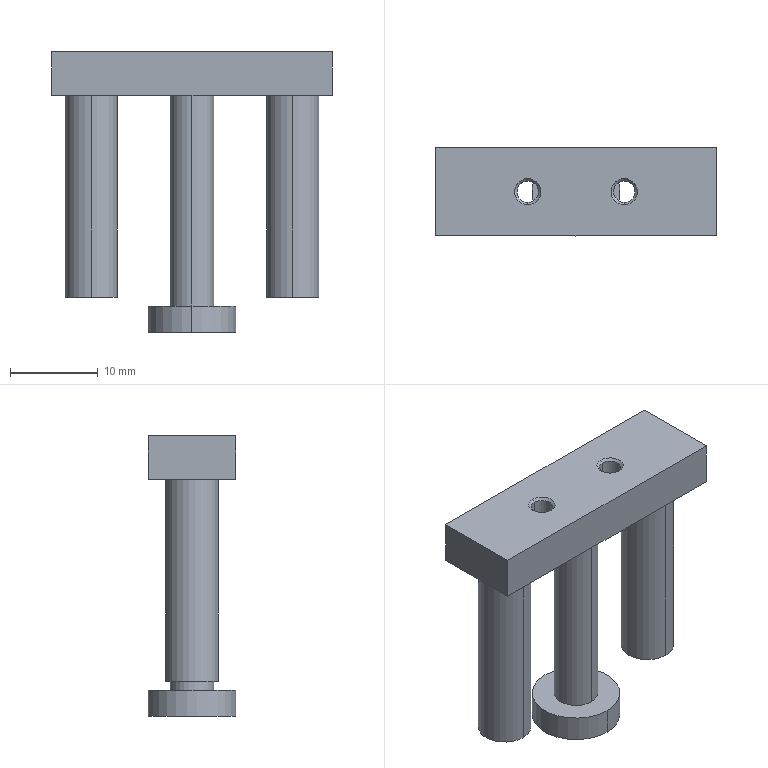Component | SolidWorks | MGJ10-15-1_2-11-1 | 1 solid | 30 faces | box 32 x 10 x 32 mm | volume 3559 mm3 | cylinder 12 | plane 10 | cone 8 | commonest cylinder face diameters 2.459 x4 6 x4 5 x2 10 x2
STEP:
#1=CARTESIAN_POINT('',(-0.4599,-4.569,-11.27));
#2=VERTEX_POINT('',#1);
#3=CARTESIAN_POINT('',(-0.4599,-4.665,-11.27));
#4=VERTEX_POINT('',#3);
#5=CARTESIAN_POINT('',(-0.4599,-4.617,-11.27));
#6=DIRECTION('',(0.,-0.,1.));
#7=DIRECTION('',(1.,0.,-0.));
#8=AXIS2_PLACEMENT_3D('',#5,#6,#7);
#9=CIRCLE('',#8,0.04841);
#10=EDGE_CURVE('',#2,#4,#9,.T.);
#11=ORIENTED_EDGE('',*,*,#10,.F.);
#12=CARTESIAN_POINT('',(-0.4599,-4.558,-11.259));
#13=VERTEX_POINT('',#12);
#14=CARTESIAN_POINT('',(-0.4599,-4.558,-11.259));
#15=DIRECTION('',(0.,0.7071,0.7071));
#16=VECTOR('',#15,39.37);
#17=LINE('',#14,#16);
#18=EDGE_CURVE('',#2,#13,#17,.T.);
#19=ORIENTED_EDGE('',*,*,#18,.T.);
#20=CARTESIAN_POINT('',(-0.4599,-4.676,-11.259));
#21=VERTEX_POINT('',#20);
#22=CARTESIAN_POINT('',(-0.4599,-4.617,-11.259));
#23=DIRECTION('',(0.,-0.,1.));
#24=DIRECTION('',(0.,-1.,0.));
#25=AXIS2_PLACEMENT_3D('',#22,#23,#24);
#26=CIRCLE('',#25,0.05906);
#27=EDGE_CURVE('',#13,#21,#26,.T.);
#28=ORIENTED_EDGE('',*,*,#27,.T.);
#29=CARTESIAN_POINT('',(-0.4599,-4.676,-11.259));
#30=DIRECTION('',(0.,-0.7071,0.7071));
#31=VECTOR('',#30,39.37);
#32=LINE('',#29,#31);
#33=EDGE_CURVE('',#4,#21,#32,.T.);
#34=ORIENTED_EDGE('',*,*,#33,.F.);
#35=EDGE_LOOP('',(#11,#19,#28,#34));
#36=FACE_OUTER_BOUND('',#35,.T.);
#37=CARTESIAN_POINT('',(-0.4599,-4.617,-11.259));
#38=DIRECTION('',(0.,-0.,1.));
#39=DIRECTION('',(0.,-1.,0.));
#40=AXIS2_PLACEMENT_3D('',#37,#38,#39);
#41=CONICAL_SURFACE('',#40,0.05906,0.7854);
#42=ADVANCED_FACE('',(#36),#41,.F.);
#43=CARTESIAN_POINT('',(-0.8929,-4.569,-11.27));
#44=VERTEX_POINT('',#43);
#45=CARTESIAN_POINT('',(-0.8929,-4.665,-11.27));
#46=VERTEX_POINT('',#45);
#47=CARTESIAN_POINT('',(-0.8929,-4.617,-11.27));
#48=DIRECTION('',(0.,-0.,1.));
#49=DIRECTION('',(1.,0.,-0.));
#50=AXIS2_PLACEMENT_3D('',#47,#48,#49);
#51=CIRCLE('',#50,0.04841);
#52=EDGE_CURVE('',#44,#46,#51,.T.);
#53=ORIENTED_EDGE('',*,*,#52,.F.);
#54=CARTESIAN_POINT('',(-0.8929,-4.558,-11.259));
#55=VERTEX_POINT('',#54);
#56=CARTESIAN_POINT('',(-0.8929,-4.558,-11.259));
#57=DIRECTION('',(0.,0.7071,0.7071));
#58=VECTOR('',#57,39.37);
#59=LINE('',#56,#58);
#60=EDGE_CURVE('',#44,#55,#59,.T.);
#61=ORIENTED_EDGE('',*,*,#60,.T.);
#62=CARTESIAN_POINT('',(-0.8929,-4.676,-11.259));
#63=VERTEX_POINT('',#62);
#64=CARTESIAN_POINT('',(-0.8929,-4.617,-11.259));
#65=DIRECTION('',(0.,-0.,1.));
#66=DIRECTION('',(0.,-1.,0.));
#67=AXIS2_PLACEMENT_3D('',#64,#65,#66);
#68=CIRCLE('',#67,0.05906);
#69=EDGE_CURVE('',#55,#63,#68,.T.);
#70=ORIENTED_EDGE('',*,*,#69,.T.);
#71=CARTESIAN_POINT('',(-0.8929,-4.676,-11.259));
#72=DIRECTION('',(0.,-0.7071,0.7071));
#73=VECTOR('',#72,39.37);
#74=LINE('',#71,#73);
#75=EDGE_CURVE('',#46,#63,#74,.T.);
#76=ORIENTED_EDGE('',*,*,#75,.F.);
#77=EDGE_LOOP('',(#53,#61,#70,#76));
#78=FACE_OUTER_BOUND('',#77,.T.);
#79=CARTESIAN_POINT('',(-0.8929,-4.617,-11.259));
#80=DIRECTION('',(0.,-0.,1.));
#81=DIRECTION('',(0.,-1.,0.));
#82=AXIS2_PLACEMENT_3D('',#79,#80,#81);
#83=CONICAL_SURFACE('',#82,0.05906,0.7854);
#84=ADVANCED_FACE('',(#78),#83,.F.);
#85=ORIENTED_EDGE('',*,*,#10,.T.);
#86=CARTESIAN_POINT('',(-0.4599,-4.665,-11.445));
#87=VERTEX_POINT('',#86);
#88=CARTESIAN_POINT('',(-0.4599,-4.665,-11.357));
#89=DIRECTION('',(-0.,0.,-1.));
#90=VECTOR('',#89,39.37);
#91=LINE('',#88,#90);
#92=EDGE_CURVE('',#4,#87,#91,.T.);
#93=ORIENTED_EDGE('',*,*,#92,.T.);
#94=CARTESIAN_POINT('',(-0.4599,-4.569,-11.445));
#95=VERTEX_POINT('',#94);
#96=CARTESIAN_POINT('',(-0.4599,-4.617,-11.445));
#97=DIRECTION('',(0.,-0.,1.));
#98=DIRECTION('',(0.,1.,0.));
#99=AXIS2_PLACEMENT_3D('',#96,#97,#98);
#100=CIRCLE('',#99,0.04841);
#101=EDGE_CURVE('',#95,#87,#100,.T.);
#102=ORIENTED_EDGE('',*,*,#101,.F.);
#103=CARTESIAN_POINT('',(-0.4599,-4.569,-11.357));
#104=DIRECTION('',(-0.,0.,-1.));
#105=VECTOR('',#104,39.37);
#106=LINE('',#103,#105);
#107=EDGE_CURVE('',#2,#95,#106,.T.);
#108=ORIENTED_EDGE('',*,*,#107,.F.);
#109=EDGE_LOOP('',(#85,#93,#102,#108));
#110=FACE_OUTER_BOUND('',#109,.T.);
#111=CARTESIAN_POINT('',(-0.4599,-4.617,-11.357));
#112=DIRECTION('',(-0.,0.,-1.));
#113=DIRECTION('',(0.,1.,0.));
#114=AXIS2_PLACEMENT_3D('',#111,#112,#113);
#115=CYLINDRICAL_SURFACE('',#114,0.04841);
#116=ADVANCED_FACE('',(#110),#115,.F.);
#117=ORIENTED_EDGE('',*,*,#52,.T.);
#118=CARTESIAN_POINT('',(-0.8929,-4.665,-11.445));
#119=VERTEX_POINT('',#118);
#120=CARTESIAN_POINT('',(-0.8929,-4.665,-11.357));
#121=DIRECTION('',(-0.,0.,-1.));
#122=VECTOR('',#121,39.37);
#123=LINE('',#120,#122);
#124=EDGE_CURVE('',#46,#119,#123,.T.);
#125=ORIENTED_EDGE('',*,*,#124,.T.);
#126=CARTESIAN_POINT('',(-0.8929,-4.569,-11.445));
#127=VERTEX_POINT('',#126);
#128=CARTESIAN_POINT('',(-0.8929,-4.617,-11.445));
#129=DIRECTION('',(0.,-0.,1.));
#130=DIRECTION('',(0.,1.,0.));
#131=AXIS2_PLACEMENT_3D('',#128,#129,#130);
#132=CIRCLE('',#131,0.04841);
#133=EDGE_CURVE('',#127,#119,#132,.T.);
#134=ORIENTED_EDGE('',*,*,#133,.F.);
#135=CARTESIAN_POINT('',(-0.8929,-4.569,-11.357));
#136=DIRECTION('',(-0.,0.,-1.));
#137=VECTOR('',#136,39.37);
#138=LINE('',#135,#137);
#139=EDGE_CURVE('',#44,#127,#138,.T.);
#140=ORIENTED_EDGE('',*,*,#139,.F.);
#141=EDGE_LOOP('',(#117,#125,#134,#140));
#142=FACE_OUTER_BOUND('',#141,.T.);
#143=CARTESIAN_POINT('',(-0.8929,-4.617,-11.357));
#144=DIRECTION('',(-0.,0.,-1.));
#145=DIRECTION('',(0.,1.,0.));
#146=AXIS2_PLACEMENT_3D('',#143,#144,#145);
#147=CYLINDRICAL_SURFACE('',#146,0.04841);
#148=ADVANCED_FACE('',(#142),#147,.F.);
#149=CARTESIAN_POINT('',(-0.2236,-4.735,-11.456));
#150=VERTEX_POINT('',#149);
#151=CARTESIAN_POINT('',(-0.2236,-4.499,-11.456));
#152=VERTEX_POINT('',#151);
#153=CARTESIAN_POINT('',(-0.2236,-4.617,-11.456));
#154=DIRECTION('',(0.,-0.,1.));
#155=DIRECTION('',(0.,1.,0.));
#156=AXIS2_PLACEMENT_3D('',#153,#154,#155);
#157=CIRCLE('',#156,0.1181);
#158=EDGE_CURVE('',#150,#152,#157,.T.);
#159=ORIENTED_EDGE('',*,*,#158,.F.);
#160=CARTESIAN_POINT('',(-0.2236,-4.735,-12.361));
#161=VERTEX_POINT('',#160);
#162=CARTESIAN_POINT('',(-0.2236,-4.735,-11.909));
#163=DIRECTION('',(-0.,0.,-1.));
#164=VECTOR('',#163,39.37);
#165=LINE('',#162,#164);
#166=EDGE_CURVE('',#150,#161,#165,.T.);
#167=ORIENTED_EDGE('',*,*,#166,.T.);
#168=CARTESIAN_POINT('',(-0.2236,-4.499,-12.361));
#169=VERTEX_POINT('',#168);
#170=CARTESIAN_POINT('',(-0.2236,-4.617,-12.361));
#171=DIRECTION('',(0.,-0.,1.));
#172=DIRECTION('',(0.,1.,0.));
#173=AXIS2_PLACEMENT_3D('',#170,#171,#172);
#174=CIRCLE('',#173,0.1181);
#175=EDGE_CURVE('',#161,#169,#174,.T.);
#176=ORIENTED_EDGE('',*,*,#175,.T.);
#177=CARTESIAN_POINT('',(-0.2236,-4.499,-11.909));
#178=DIRECTION('',(-0.,0.,-1.));
#179=VECTOR('',#178,39.37);
#180=LINE('',#177,#179);
#181=EDGE_CURVE('',#152,#169,#180,.T.);
#182=ORIENTED_EDGE('',*,*,#181,.F.);
#183=EDGE_LOOP('',(#159,#167,#176,#182));
#184=FACE_OUTER_BOUND('',#183,.T.);
#185=CARTESIAN_POINT('',(-0.2236,-4.617,-11.909));
#186=DIRECTION('',(-0.,0.,-1.));
#187=DIRECTION('',(0.,1.,0.));
#188=AXIS2_PLACEMENT_3D('',#185,#186,#187);
#189=CYLINDRICAL_SURFACE('',#188,0.1181);
#190=ADVANCED_FACE('',(#184),#189,.T.);
#191=CARTESIAN_POINT('',(-1.129,-4.735,-11.456));
#192=VERTEX_POINT('',#191);
#193=CARTESIAN_POINT('',(-1.129,-4.499,-11.456));
#194=VERTEX_POINT('',#193);
#195=CARTESIAN_POINT('',(-1.129,-4.617,-11.456));
#196=DIRECTION('',(0.,-0.,1.));
#197=DIRECTION('',(0.,1.,0.));
#198=AXIS2_PLACEMENT_3D('',#195,#196,#197);
#199=CIRCLE('',#198,0.1181);
#200=EDGE_CURVE('',#192,#194,#199,.T.);
#201=ORIENTED_EDGE('',*,*,#200,.F.);
#202=CARTESIAN_POINT('',(-1.129,-4.735,-12.361));
#203=VERTEX_POINT('',#202);
#204=CARTESIAN_POINT('',(-1.129,-4.735,-11.909));
#205=DIRECTION('',(-0.,0.,-1.));
#206=VECTOR('',#205,39.37);
#207=LINE('',#204,#206);
#208=EDGE_CURVE('',#192,#203,#207,.T.);
#209=ORIENTED_EDGE('',*,*,#208,.T.);
#210=CARTESIAN_POINT('',(-1.129,-4.499,-12.361));
#211=VERTEX_POINT('',#210);
#212=CARTESIAN_POINT('',(-1.129,-4.617,-12.361));
#213=DIRECTION('',(0.,-0.,1.));
#214=DIRECTION('',(0.,1.,0.));
#215=AXIS2_PLACEMENT_3D('',#212,#213,#214);
#216=CIRCLE('',#215,0.1181);
#217=EDGE_CURVE('',#203,#211,#216,.T.);
#218=ORIENTED_EDGE('',*,*,#217,.T.);
#219=CARTESIAN_POINT('',(-1.129,-4.499,-11.909));
#220=DIRECTION('',(-0.,0.,-1.));
#221=VECTOR('',#220,39.37);
#222=LINE('',#219,#221);
#223=EDGE_CURVE('',#194,#211,#222,.T.);
#224=ORIENTED_EDGE('',*,*,#223,.F.);
#225=EDGE_LOOP('',(#201,#209,#218,#224));
#226=FACE_OUTER_BOUND('',#225,.T.);
#227=CARTESIAN_POINT('',(-1.129,-4.617,-11.909));
#228=DIRECTION('',(-0.,0.,-1.));
#229=DIRECTION('',(0.,1.,0.));
#230=AXIS2_PLACEMENT_3D('',#227,#228,#229);
#231=CYLINDRICAL_SURFACE('',#230,0.1181);
#232=ADVANCED_FACE('',(#226),#231,.T.);
#233=CARTESIAN_POINT('',(-0.6764,-4.715,-11.456));
#234=VERTEX_POINT('',#233);
#235=CARTESIAN_POINT('',(-0.6764,-4.519,-11.456));
#236=VERTEX_POINT('',#235);
#237=CARTESIAN_POINT('',(-0.6764,-4.617,-11.456));
#238=DIRECTION('',(0.,-0.,1.));
#239=DIRECTION('',(0.,1.,0.));
#240=AXIS2_PLACEMENT_3D('',#237,#238,#239);
#241=CIRCLE('',#240,0.09843);
#242=EDGE_CURVE('',#234,#236,#241,.T.);
#243=ORIENTED_EDGE('',*,*,#242,.F.);
#244=CARTESIAN_POINT('',(-0.6764,-4.715,-12.401));
#245=VERTEX_POINT('',#244);
#246=CARTESIAN_POINT('',(-0.6764,-4.715,-11.928));
#247=DIRECTION('',(-0.,0.,-1.));
#248=VECTOR('',#247,39.37);
#249=LINE('',#246,#248);
#250=EDGE_CURVE('',#234,#245,#249,.T.);
#251=ORIENTED_EDGE('',*,*,#250,.T.);
#252=CARTESIAN_POINT('',(-0.6764,-4.519,-12.401));
#253=VERTEX_POINT('',#252);
#254=CARTESIAN_POINT('',(-0.6764,-4.617,-12.401));
#255=DIRECTION('',(0.,-0.,1.));
#256=DIRECTION('',(0.,1.,0.));
#257=AXIS2_PLACEMENT_3D('',#254,#255,#256);
#258=CIRCLE('',#257,0.09843);
#259=EDGE_CURVE('',#245,#253,#258,.T.);
#260=ORIENTED_EDGE('',*,*,#259,.T.);
#261=CARTESIAN_POINT('',(-0.6764,-4.519,-11.928));
#262=DIRECTION('',(-0.,0.,-1.));
#263=VECTOR('',#262,39.37);
#264=LINE('',#261,#263);
#265=EDGE_CURVE('',#236,#253,#264,.T.);
#266=ORIENTED_EDGE('',*,*,#265,.F.);
#267=EDGE_LOOP('',(#243,#251,#260,#266));
#268=FACE_OUTER_BOUND('',#267,.T.);
#269=CARTESIAN_POINT('',(-0.6764,-4.617,-11.928));
#270=DIRECTION('',(-0.,0.,-1.));
#271=DIRECTION('',(0.,1.,0.));
#272=AXIS2_PLACEMENT_3D('',#269,#270,#271);
#273=CYLINDRICAL_SURFACE('',#272,0.09843);
#274=ADVANCED_FACE('',(#268),#273,.T.);
#275=ORIENTED_EDGE('',*,*,#101,.T.);
#276=CARTESIAN_POINT('',(-0.4599,-4.676,-11.456));
#277=VERTEX_POINT('',#276);
#278=CARTESIAN_POINT('',(-0.4599,-4.676,-11.456));
#279=DIRECTION('',(-0.,-0.7071,-0.7071));
#280=VECTOR('',#279,39.37);
#281=LINE('',#278,#280);
#282=EDGE_CURVE('',#87,#277,#281,.T.);
#283=ORIENTED_EDGE('',*,*,#282,.T.);
#284=CARTESIAN_POINT('',(-0.4599,-4.558,-11.456));
#285=VERTEX_POINT('',#284);
#286=CARTESIAN_POINT('',(-0.4599,-4.617,-11.456));
#287=DIRECTION('',(0.,-0.,1.));
#288=DIRECTION('',(0.,1.,0.));
#289=AXIS2_PLACEMENT_3D('',#286,#287,#288);
#290=CIRCLE('',#289,0.05906);
#291=EDGE_CURVE('',#285,#277,#290,.T.);
#292=ORIENTED_EDGE('',*,*,#291,.F.);
#293=CARTESIAN_POINT('',(-0.4599,-4.558,-11.456));
#294=DIRECTION('',(-0.,0.7071,-0.7071));
#295=VECTOR('',#294,39.37);
#296=LINE('',#293,#295);
#297=EDGE_CURVE('',#95,#285,#296,.T.);
#298=ORIENTED_EDGE('',*,*,#297,.F.);
#299=EDGE_LOOP('',(#275,#283,#292,#298));
#300=FACE_OUTER_BOUND('',#299,.T.);
#301=CARTESIAN_POINT('',(-0.4599,-4.617,-11.456));
#302=DIRECTION('',(-0.,0.,-1.));
#303=DIRECTION('',(0.,1.,0.));
#304=AXIS2_PLACEMENT_3D('',#301,#302,#303);
#305=CONICAL_SURFACE('',#304,0.05906,0.7854);
#306=ADVANCED_FACE('',(#300),#305,.F.);
#307=ORIENTED_EDGE('',*,*,#133,.T.);
#308=CARTESIAN_POINT('',(-0.8929,-4.676,-11.456));
#309=VERTEX_POINT('',#308);
#310=CARTESIAN_POINT('',(-0.8929,-4.676,-11.456));
#311=DIRECTION('',(-0.,-0.7071,-0.7071));
#312=VECTOR('',#311,39.37);
#313=LINE('',#310,#312);
#314=EDGE_CURVE('',#119,#309,#313,.T.);
#315=ORIENTED_EDGE('',*,*,#314,.T.);
#316=CARTESIAN_POINT('',(-0.8929,-4.558,-11.456));
#317=VERTEX_POINT('',#316);
#318=CARTESIAN_POINT('',(-0.8929,-4.617,-11.456));
#319=DIRECTION('',(0.,-0.,1.));
#320=DIRECTION('',(0.,1.,0.));
#321=AXIS2_PLACEMENT_3D('',#318,#319,#320);
#322=CIRCLE('',#321,0.05906);
#323=EDGE_CURVE('',#317,#309,#322,.T.);
#324=ORIENTED_EDGE('',*,*,#323,.F.);
#325=CARTESIAN_POINT('',(-0.8929,-4.558,-11.456));
#326=DIRECTION('',(-0.,0.7071,-0.7071));
#327=VECTOR('',#326,39.37);
#328=LINE('',#325,#327);
#329=EDGE_CURVE('',#127,#317,#328,.T.);
#330=ORIENTED_EDGE('',*,*,#329,.F.);
#331=EDGE_LOOP('',(#307,#315,#324,#330));
#332=FACE_OUTER_BOUND('',#331,.T.);
#333=CARTESIAN_POINT('',(-0.8929,-4.617,-11.456));
#334=DIRECTION('',(-0.,0.,-1.));
#335=DIRECTION('',(0.,1.,0.));
#336=AXIS2_PLACEMENT_3D('',#333,#334,#335);
#337=CONICAL_SURFACE('',#336,0.05906,0.7854);
#338=ADVANCED_FACE('',(#332),#337,.F.);
#339=CARTESIAN_POINT('',(-0.6764,-4.814,-12.401));
#340=VERTEX_POINT('',#339);
#341=CARTESIAN_POINT('',(-0.6764,-4.42,-12.401));
#342=VERTEX_POINT('',#341);
#343=CARTESIAN_POINT('',(-0.6764,-4.617,-12.401));
#344=DIRECTION('',(0.,-0.,1.));
#345=DIRECTION('',(0.,1.,0.));
#346=AXIS2_PLACEMENT_3D('',#343,#344,#345);
#347=CIRCLE('',#346,0.1969);
#348=EDGE_CURVE('',#340,#342,#347,.T.);
#349=ORIENTED_EDGE('',*,*,#348,.F.);
#350=CARTESIAN_POINT('',(-0.6764,-4.814,-12.519));
#351=VERTEX_POINT('',#350);
#352=CARTESIAN_POINT('',(-0.6764,-4.814,-12.46));
#353=DIRECTION('',(-0.,0.,-1.));
#354=VECTOR('',#353,39.37);
#355=LINE('',#352,#354);
#356=EDGE_CURVE('',#340,#351,#355,.T.);
#357=ORIENTED_EDGE('',*,*,#356,.T.);
#358=CARTESIAN_POINT('',(-0.6764,-4.42,-12.519));
#359=VERTEX_POINT('',#358);
#360=CARTESIAN_POINT('',(-0.6764,-4.617,-12.519));
#361=DIRECTION('',(0.,-0.,1.));
#362=DIRECTION('',(0.,1.,0.));
#363=AXIS2_PLACEMENT_3D('',#360,#361,#362);
#364=CIRCLE('',#363,0.1969);
#365=EDGE_CURVE('',#351,#359,#364,.T.);
#366=ORIENTED_EDGE('',*,*,#365,.T.);
#367=CARTESIAN_POINT('',(-0.6764,-4.42,-12.46));
#368=DIRECTION('',(-0.,0.,-1.));
#369=VECTOR('',#368,39.37);
#370=LINE('',#367,#369);
#371=EDGE_CURVE('',#342,#359,#370,.T.);
#372=ORIENTED_EDGE('',*,*,#371,.F.);
#373=EDGE_LOOP('',(#349,#357,#366,#372));
#374=FACE_OUTER_BOUND('',#373,.T.);
#375=CARTESIAN_POINT('',(-0.6764,-4.617,-12.46));
#376=DIRECTION('',(-0.,0.,-1.));
#377=DIRECTION('',(0.,1.,0.));
#378=AXIS2_PLACEMENT_3D('',#375,#376,#377);
#379=CYLINDRICAL_SURFACE('',#378,0.1969);
#380=ADVANCED_FACE('',(#374),#379,.T.);
#381=CARTESIAN_POINT('',(-1.306,-4.814,-11.259));
#382=VERTEX_POINT('',#381);
#383=CARTESIAN_POINT('',(-1.306,-4.42,-11.259));
#384=VERTEX_POINT('',#383);
#385=CARTESIAN_POINT('',(-1.306,-4.617,-11.259));
#386=DIRECTION('',(0.,1.,0.));
#387=VECTOR('',#386,39.37);
#388=LINE('',#385,#387);
#389=EDGE_CURVE('',#382,#384,#388,.T.);
#390=ORIENTED_EDGE('',*,*,#389,.F.);
#391=CARTESIAN_POINT('',(-0.04648,-4.814,-11.259));
#392=VERTEX_POINT('',#391);
#393=CARTESIAN_POINT('',(-0.6764,-4.814,-11.259));
#394=DIRECTION('',(-1.,0.,0.));
#395=VECTOR('',#394,39.37);
#396=LINE('',#393,#395);
#397=EDGE_CURVE('',#392,#382,#396,.T.);
#398=ORIENTED_EDGE('',*,*,#397,.F.);
#399=CARTESIAN_POINT('',(-0.04648,-4.42,-11.259));
#400=VERTEX_POINT('',#399);
#401=CARTESIAN_POINT('',(-0.04648,-4.617,-11.259));
#402=DIRECTION('',(-0.,-1.,-0.));
#403=VECTOR('',#402,39.37);
#404=LINE('',#401,#403);
#405=EDGE_CURVE('',#400,#392,#404,.T.);
#406=ORIENTED_EDGE('',*,*,#405,.F.);
#407=CARTESIAN_POINT('',(-0.6764,-4.42,-11.259));
#408=DIRECTION('',(1.,-0.,-0.));
#409=VECTOR('',#408,39.37);
#410=LINE('',#407,#409);
#411=EDGE_CURVE('',#384,#400,#410,.T.);
#412=ORIENTED_EDGE('',*,*,#411,.F.);
#413=EDGE_LOOP('',(#390,#398,#406,#412));
#414=FACE_OUTER_BOUND('',#413,.T.);
#415=CARTESIAN_POINT('',(-0.4599,-4.617,-11.259));
#416=DIRECTION('',(0.,-0.,1.));
#417=DIRECTION('',(0.,-1.,0.));
#418=AXIS2_PLACEMENT_3D('',#415,#416,#417);
#419=CIRCLE('',#418,0.05906);
#420=EDGE_CURVE('',#21,#13,#419,.T.);
#421=ORIENTED_EDGE('',*,*,#420,.F.);
#422=ORIENTED_EDGE('',*,*,#27,.F.);
#423=EDGE_LOOP('',(#421,#422));
#424=FACE_BOUND('',#423,.T.);
#425=CARTESIAN_POINT('',(-0.8929,-4.617,-11.259));
#426=DIRECTION('',(0.,-0.,1.));
#427=DIRECTION('',(0.,-1.,0.));
#428=AXIS2_PLACEMENT_3D('',#425,#426,#427);
#429=CIRCLE('',#428,0.05906);
#430=EDGE_CURVE('',#63,#55,#429,.T.);
#431=ORIENTED_EDGE('',*,*,#430,.F.);
#432=ORIENTED_EDGE('',*,*,#69,.F.);
#433=EDGE_LOOP('',(#431,#432));
#434=FACE_BOUND('',#433,.T.);
#435=CARTESIAN_POINT('',(-0.6764,-4.617,-11.259));
#436=DIRECTION('',(-0.,0.,-1.));
#437=DIRECTION('',(0.,1.,0.));
#438=AXIS2_PLACEMENT_3D('',#435,#436,#437);
#439=PLANE('',#438);
#440=ADVANCED_FACE('',(#414,#424,#434),#439,.F.);
#441=CARTESIAN_POINT('',(-0.04648,-4.42,-11.456));
#442=VERTEX_POINT('',#441);
#443=CARTESIAN_POINT('',(-1.306,-4.42,-11.456));
#444=VERTEX_POINT('',#443);
#445=CARTESIAN_POINT('',(-1.306,-4.42,-11.456));
#446=DIRECTION('',(-1.,0.,0.));
#447=VECTOR('',#446,39.37);
#448=LINE('',#445,#447);
#449=EDGE_CURVE('',#442,#444,#448,.T.);
#450=ORIENTED_EDGE('',*,*,#449,.T.);
#451=CARTESIAN_POINT('',(-1.306,-4.42,-11.456));
#452=DIRECTION('',(0.,-0.,1.));
#453=VECTOR('',#452,39.37);
#454=LINE('',#451,#453);
#455=EDGE_CURVE('',#444,#384,#454,.T.);
#456=ORIENTED_EDGE('',*,*,#455,.T.);
#457=ORIENTED_EDGE('',*,*,#411,.T.);
#458=CARTESIAN_POINT('',(-0.04648,-4.42,-11.456));
#459=DIRECTION('',(-0.,0.,-1.));
#460=VECTOR('',#459,39.37);
#461=LINE('',#458,#460);
#462=EDGE_CURVE('',#400,#442,#461,.T.);
#463=ORIENTED_EDGE('',*,*,#462,.T.);
#464=EDGE_LOOP('',(#450,#456,#457,#463));
#465=FACE_OUTER_BOUND('',#464,.T.);
#466=CARTESIAN_POINT('',(-1.306,-4.42,-11.456));
#467=DIRECTION('',(0.,1.,0.));
#468=DIRECTION('',(0.,-0.,1.));
#469=AXIS2_PLACEMENT_3D('',#466,#467,#468);
#470=PLANE('',#469);
#471=ADVANCED_FACE('',(#465),#470,.T.);
#472=CARTESIAN_POINT('',(-1.306,-4.814,-11.456));
#473=VERTEX_POINT('',#472);
#474=CARTESIAN_POINT('',(-1.306,-4.814,-11.456));
#475=DIRECTION('',(-0.,-1.,-0.));
#476=VECTOR('',#475,39.37);
#477=LINE('',#474,#476);
#478=EDGE_CURVE('',#444,#473,#477,.T.);
#479=ORIENTED_EDGE('',*,*,#478,.T.);
#480=CARTESIAN_POINT('',(-1.306,-4.814,-11.456));
#481=DIRECTION('',(0.,-0.,1.));
#482=VECTOR('',#481,39.37);
#483=LINE('',#480,#482);
#484=EDGE_CURVE('',#473,#382,#483,.T.);
#485=ORIENTED_EDGE('',*,*,#484,.T.);
#486=ORIENTED_EDGE('',*,*,#389,.T.);
#487=ORIENTED_EDGE('',*,*,#455,.F.);
#488=EDGE_LOOP('',(#479,#485,#486,#487));
#489=FACE_OUTER_BOUND('',#488,.T.);
#490=CARTESIAN_POINT('',(-1.306,-4.814,-11.456));
#491=DIRECTION('',(-1.,0.,0.));
#492=DIRECTION('',(0.,1.,0.));
#493=AXIS2_PLACEMENT_3D('',#490,#491,#492);
#494=PLANE('',#493);
#495=ADVANCED_FACE('',(#489),#494,.T.);
#496=CARTESIAN_POINT('',(-0.04648,-4.814,-11.456));
#497=VERTEX_POINT('',#496);
#498=CARTESIAN_POINT('',(-0.04648,-4.814,-11.456));
#499=DIRECTION('',(1.,-0.,-0.));
#500=VECTOR('',#499,39.37);
#501=LINE('',#498,#500);
#502=EDGE_CURVE('',#473,#497,#501,.T.);
#503=ORIENTED_EDGE('',*,*,#502,.T.);
#504=CARTESIAN_POINT('',(-0.04648,-4.814,-11.456));
#505=DIRECTION('',(0.,-0.,1.));
#506=VECTOR('',#505,39.37);
#507=LINE('',#504,#506);
#508=EDGE_CURVE('',#497,#392,#507,.T.);
#509=ORIENTED_EDGE('',*,*,#508,.T.);
#510=ORIENTED_EDGE('',*,*,#397,.T.);
#511=ORIENTED_EDGE('',*,*,#484,.F.);
#512=EDGE_LOOP('',(#503,#509,#510,#511));
#513=FACE_OUTER_BOUND('',#512,.T.);
#514=CARTESIAN_POINT('',(-0.04648,-4.814,-11.456));
#515=DIRECTION('',(-0.,-1.,-0.));
#516=DIRECTION('',(-0.,0.,-1.));
#517=AXIS2_PLACEMENT_3D('',#514,#515,#516);
#518=PLANE('',#517);
#519=ADVANCED_FACE('',(#513),#518,.T.);
#520=CARTESIAN_POINT('',(-0.04648,-4.42,-11.456));
#521=DIRECTION('',(0.,1.,0.));
#522=VECTOR('',#521,39.37);
#523=LINE('',#520,#522);
#524=EDGE_CURVE('',#497,#442,#523,.T.);
#525=ORIENTED_EDGE('',*,*,#524,.T.);
#526=ORIENTED_EDGE('',*,*,#462,.F.);
#527=ORIENTED_EDGE('',*,*,#405,.T.);
#528=ORIENTED_EDGE('',*,*,#508,.F.);
#529=EDGE_LOOP('',(#525,#526,#527,#528));
#530=FACE_OUTER_BOUND('',#529,.T.);
#531=CARTESIAN_POINT('',(-0.04648,-4.42,-11.456));
#532=DIRECTION('',(1.,-0.,-0.));
#533=DIRECTION('',(-0.,-1.,-0.));
#534=AXIS2_PLACEMENT_3D('',#531,#532,#533);
#535=PLANE('',#534);
#536=ADVANCED_FACE('',(#530),#535,.T.);
#537=ORIENTED_EDGE('',*,*,#18,.F.);
#538=CARTESIAN_POINT('',(-0.4599,-4.617,-11.27));
#539=DIRECTION('',(0.,-0.,1.));
#540=DIRECTION('',(1.,0.,-0.));
#541=AXIS2_PLACEMENT_3D('',#538,#539,#540);
#542=CIRCLE('',#541,0.04841);
#543=EDGE_CURVE('',#4,#2,#542,.T.);
#544=ORIENTED_EDGE('',*,*,#543,.F.);
#545=ORIENTED_EDGE('',*,*,#33,.T.);
#546=ORIENTED_EDGE('',*,*,#420,.T.);
#547=EDGE_LOOP('',(#537,#544,#545,#546));
#548=FACE_OUTER_BOUND('',#547,.T.);
#549=CARTESIAN_POINT('',(-0.4599,-4.617,-11.259));
#550=DIRECTION('',(0.,-0.,1.));
#551=DIRECTION('',(0.,-1.,0.));
#552=AXIS2_PLACEMENT_3D('',#549,#550,#551);
#553=CONICAL_SURFACE('',#552,0.05906,0.7854);
#554=ADVANCED_FACE('',(#548),#553,.F.);
#555=ORIENTED_EDGE('',*,*,#60,.F.);
#556=CARTESIAN_POINT('',(-0.8929,-4.617,-11.27));
#557=DIRECTION('',(0.,-0.,1.));
#558=DIRECTION('',(1.,0.,-0.));
#559=AXIS2_PLACEMENT_3D('',#556,#557,#558);
#560=CIRCLE('',#559,0.04841);
#561=EDGE_CURVE('',#46,#44,#560,.T.);
#562=ORIENTED_EDGE('',*,*,#561,.F.);
#563=ORIENTED_EDGE('',*,*,#75,.T.);
#564=ORIENTED_EDGE('',*,*,#430,.T.);
#565=EDGE_LOOP('',(#555,#562,#563,#564));
#566=FACE_OUTER_BOUND('',#565,.T.);
#567=CARTESIAN_POINT('',(-0.8929,-4.617,-11.259));
#568=DIRECTION('',(0.,-0.,1.));
#569=DIRECTION('',(0.,-1.,0.));
#570=AXIS2_PLACEMENT_3D('',#567,#568,#569);
#571=CONICAL_SURFACE('',#570,0.05906,0.7854);
#572=ADVANCED_FACE('',(#566),#571,.F.);
#573=ORIENTED_EDGE('',*,*,#524,.F.);
#574=ORIENTED_EDGE('',*,*,#502,.F.);
#575=ORIENTED_EDGE('',*,*,#478,.F.);
#576=ORIENTED_EDGE('',*,*,#449,.F.);
#577=EDGE_LOOP('',(#573,#574,#575,#576));
#578=FACE_OUTER_BOUND('',#577,.T.);
#579=CARTESIAN_POINT('',(-0.2236,-4.617,-11.456));
#580=DIRECTION('',(0.,-0.,1.));
#581=DIRECTION('',(0.,1.,0.));
#582=AXIS2_PLACEMENT_3D('',#579,#580,#581);
#583=CIRCLE('',#582,0.1181);
#584=EDGE_CURVE('',#152,#150,#583,.T.);
#585=ORIENTED_EDGE('',*,*,#584,.T.);
#586=ORIENTED_EDGE('',*,*,#158,.T.);
#587=EDGE_LOOP('',(#585,#586));
#588=FACE_BOUND('',#587,.T.);
#589=CARTESIAN_POINT('',(-1.129,-4.617,-11.456));
#590=DIRECTION('',(0.,-0.,1.));
#591=DIRECTION('',(0.,1.,0.));
#592=AXIS2_PLACEMENT_3D('',#589,#590,#591);
#593=CIRCLE('',#592,0.1181);
#594=EDGE_CURVE('',#194,#192,#593,.T.);
#595=ORIENTED_EDGE('',*,*,#594,.T.);
#596=ORIENTED_EDGE('',*,*,#200,.T.);
#597=EDGE_LOOP('',(#595,#596));
#598=FACE_BOUND('',#597,.T.);
#599=CARTESIAN_POINT('',(-0.6764,-4.617,-11.456));
#600=DIRECTION('',(0.,-0.,1.));
#601=DIRECTION('',(0.,1.,0.));
#602=AXIS2_PLACEMENT_3D('',#599,#600,#601);
#603=CIRCLE('',#602,0.09843);
#604=EDGE_CURVE('',#236,#234,#603,.T.);
#605=ORIENTED_EDGE('',*,*,#604,.T.);
#606=ORIENTED_EDGE('',*,*,#242,.T.);
#607=EDGE_LOOP('',(#605,#606));
#608=FACE_BOUND('',#607,.T.);
#609=ORIENTED_EDGE('',*,*,#291,.T.);
#610=CARTESIAN_POINT('',(-0.4599,-4.617,-11.456));
#611=DIRECTION('',(0.,-0.,1.));
#612=DIRECTION('',(0.,1.,0.));
#613=AXIS2_PLACEMENT_3D('',#610,#611,#612);
#614=CIRCLE('',#613,0.05906);
#615=EDGE_CURVE('',#277,#285,#614,.T.);
#616=ORIENTED_EDGE('',*,*,#615,.T.);
#617=EDGE_LOOP('',(#609,#616));
#618=FACE_BOUND('',#617,.T.);
#619=ORIENTED_EDGE('',*,*,#323,.T.);
#620=CARTESIAN_POINT('',(-0.8929,-4.617,-11.456));
#621=DIRECTION('',(0.,-0.,1.));
#622=DIRECTION('',(0.,1.,0.));
#623=AXIS2_PLACEMENT_3D('',#620,#621,#622);
#624=CIRCLE('',#623,0.05906);
#625=EDGE_CURVE('',#309,#317,#624,.T.);
#626=ORIENTED_EDGE('',*,*,#625,.T.);
#627=EDGE_LOOP('',(#619,#626));
#628=FACE_BOUND('',#627,.T.);
#629=CARTESIAN_POINT('',(-0.6764,-4.617,-11.456));
#630=DIRECTION('',(-0.,0.,-1.));
#631=DIRECTION('',(0.,1.,0.));
#632=AXIS2_PLACEMENT_3D('',#629,#630,#631);
#633=PLANE('',#632);
#634=ADVANCED_FACE('',(#578,#588,#598,#608,#618,#628),#633,.T.);
#635=ORIENTED_EDGE('',*,*,#92,.F.);
#636=ORIENTED_EDGE('',*,*,#543,.T.);
#637=ORIENTED_EDGE('',*,*,#107,.T.);
#638=CARTESIAN_POINT('',(-0.4599,-4.617,-11.445));
#639=DIRECTION('',(0.,-0.,1.));
#640=DIRECTION('',(0.,1.,0.));
#641=AXIS2_PLACEMENT_3D('',#638,#639,#640);
#642=CIRCLE('',#641,0.04841);
#643=EDGE_CURVE('',#87,#95,#642,.T.);
#644=ORIENTED_EDGE('',*,*,#643,.F.);
#645=EDGE_LOOP('',(#635,#636,#637,#644));
#646=FACE_OUTER_BOUND('',#645,.T.);
#647=CARTESIAN_POINT('',(-0.4599,-4.617,-11.357));
#648=DIRECTION('',(-0.,0.,-1.));
#649=DIRECTION('',(0.,1.,0.));
#650=AXIS2_PLACEMENT_3D('',#647,#648,#649);
#651=CYLINDRICAL_SURFACE('',#650,0.04841);
#652=ADVANCED_FACE('',(#646),#651,.F.);
#653=ORIENTED_EDGE('',*,*,#124,.F.);
#654=ORIENTED_EDGE('',*,*,#561,.T.);
#655=ORIENTED_EDGE('',*,*,#139,.T.);
#656=CARTESIAN_POINT('',(-0.8929,-4.617,-11.445));
#657=DIRECTION('',(0.,-0.,1.));
#658=DIRECTION('',(0.,1.,0.));
#659=AXIS2_PLACEMENT_3D('',#656,#657,#658);
#660=CIRCLE('',#659,0.04841);
#661=EDGE_CURVE('',#119,#127,#660,.T.);
#662=ORIENTED_EDGE('',*,*,#661,.F.);
#663=EDGE_LOOP('',(#653,#654,#655,#662));
#664=FACE_OUTER_BOUND('',#663,.T.);
#665=CARTESIAN_POINT('',(-0.8929,-4.617,-11.357));
#666=DIRECTION('',(-0.,0.,-1.));
#667=DIRECTION('',(0.,1.,0.));
#668=AXIS2_PLACEMENT_3D('',#665,#666,#667);
#669=CYLINDRICAL_SURFACE('',#668,0.04841);
#670=ADVANCED_FACE('',(#664),#669,.F.);
#671=ORIENTED_EDGE('',*,*,#166,.F.);
#672=ORIENTED_EDGE('',*,*,#584,.F.);
#673=ORIENTED_EDGE('',*,*,#181,.T.);
#674=CARTESIAN_POINT('',(-0.2236,-4.617,-12.361));
#675=DIRECTION('',(0.,-0.,1.));
#676=DIRECTION('',(0.,1.,0.));
#677=AXIS2_PLACEMENT_3D('',#674,#675,#676);
#678=CIRCLE('',#677,0.1181);
#679=EDGE_CURVE('',#169,#161,#678,.T.);
#680=ORIENTED_EDGE('',*,*,#679,.T.);
#681=EDGE_LOOP('',(#671,#672,#673,#680));
#682=FACE_OUTER_BOUND('',#681,.T.);
#683=CARTESIAN_POINT('',(-0.2236,-4.617,-11.909));
#684=DIRECTION('',(-0.,0.,-1.));
#685=DIRECTION('',(0.,1.,0.));
#686=AXIS2_PLACEMENT_3D('',#683,#684,#685);
#687=CYLINDRICAL_SURFACE('',#686,0.1181);
#688=ADVANCED_FACE('',(#682),#687,.T.);
#689=ORIENTED_EDGE('',*,*,#208,.F.);
#690=ORIENTED_EDGE('',*,*,#594,.F.);
#691=ORIENTED_EDGE('',*,*,#223,.T.);
#692=CARTESIAN_POINT('',(-1.129,-4.617,-12.361));
#693=DIRECTION('',(0.,-0.,1.));
#694=DIRECTION('',(0.,1.,0.));
#695=AXIS2_PLACEMENT_3D('',#692,#693,#694);
#696=CIRCLE('',#695,0.1181);
#697=EDGE_CURVE('',#211,#203,#696,.T.);
#698=ORIENTED_EDGE('',*,*,#697,.T.);
#699=EDGE_LOOP('',(#689,#690,#691,#698));
#700=FACE_OUTER_BOUND('',#699,.T.);
#701=CARTESIAN_POINT('',(-1.129,-4.617,-11.909));
#702=DIRECTION('',(-0.,0.,-1.));
#703=DIRECTION('',(0.,1.,0.));
#704=AXIS2_PLACEMENT_3D('',#701,#702,#703);
#705=CYLINDRICAL_SURFACE('',#704,0.1181);
#706=ADVANCED_FACE('',(#700),#705,.T.);
#707=ORIENTED_EDGE('',*,*,#250,.F.);
#708=ORIENTED_EDGE('',*,*,#604,.F.);
#709=ORIENTED_EDGE('',*,*,#265,.T.);
#710=CARTESIAN_POINT('',(-0.6764,-4.617,-12.401));
#711=DIRECTION('',(0.,-0.,1.));
#712=DIRECTION('',(0.,1.,0.));
#713=AXIS2_PLACEMENT_3D('',#710,#711,#712);
#714=CIRCLE('',#713,0.09843);
#715=EDGE_CURVE('',#253,#245,#714,.T.);
#716=ORIENTED_EDGE('',*,*,#715,.T.);
#717=EDGE_LOOP('',(#707,#708,#709,#716));
#718=FACE_OUTER_BOUND('',#717,.T.);
#719=CARTESIAN_POINT('',(-0.6764,-4.617,-11.928));
#720=DIRECTION('',(-0.,0.,-1.));
#721=DIRECTION('',(0.,1.,0.));
#722=AXIS2_PLACEMENT_3D('',#719,#720,#721);
#723=CYLINDRICAL_SURFACE('',#722,0.09843);
#724=ADVANCED_FACE('',(#718),#723,.T.);
#725=ORIENTED_EDGE('',*,*,#282,.F.);
#726=ORIENTED_EDGE('',*,*,#643,.T.);
#727=ORIENTED_EDGE('',*,*,#297,.T.);
#728=ORIENTED_EDGE('',*,*,#615,.F.);
#729=EDGE_LOOP('',(#725,#726,#727,#728));
#730=FACE_OUTER_BOUND('',#729,.T.);
#731=CARTESIAN_POINT('',(-0.4599,-4.617,-11.456));
#732=DIRECTION('',(-0.,0.,-1.));
#733=DIRECTION('',(0.,1.,0.));
#734=AXIS2_PLACEMENT_3D('',#731,#732,#733);
#735=CONICAL_SURFACE('',#734,0.05906,0.7854);
#736=ADVANCED_FACE('',(#730),#735,.F.);
#737=ORIENTED_EDGE('',*,*,#314,.F.);
#738=ORIENTED_EDGE('',*,*,#661,.T.);
#739=ORIENTED_EDGE('',*,*,#329,.T.);
#740=ORIENTED_EDGE('',*,*,#625,.F.);
#741=EDGE_LOOP('',(#737,#738,#739,#740));
#742=FACE_OUTER_BOUND('',#741,.T.);
#743=CARTESIAN_POINT('',(-0.8929,-4.617,-11.456));
#744=DIRECTION('',(-0.,0.,-1.));
#745=DIRECTION('',(0.,1.,0.));
#746=AXIS2_PLACEMENT_3D('',#743,#744,#745);
#747=CONICAL_SURFACE('',#746,0.05906,0.7854);
#748=ADVANCED_FACE('',(#742),#747,.F.);
#749=ORIENTED_EDGE('',*,*,#679,.F.);
#750=ORIENTED_EDGE('',*,*,#175,.F.);
#751=EDGE_LOOP('',(#749,#750));
#752=FACE_OUTER_BOUND('',#751,.T.);
#753=CARTESIAN_POINT('',(-0.1646,-4.617,-12.361));
#754=DIRECTION('',(-0.,0.,-1.));
#755=DIRECTION('',(0.,1.,0.));
#756=AXIS2_PLACEMENT_3D('',#753,#754,#755);
#757=PLANE('',#756);
#758=ADVANCED_FACE('',(#752),#757,.T.);
#759=ORIENTED_EDGE('',*,*,#697,.F.);
#760=ORIENTED_EDGE('',*,*,#217,.F.);
#761=EDGE_LOOP('',(#759,#760));
#762=FACE_OUTER_BOUND('',#761,.T.);
#763=CARTESIAN_POINT('',(-1.07,-4.617,-12.361));
#764=DIRECTION('',(-0.,0.,-1.));
#765=DIRECTION('',(0.,1.,0.));
#766=AXIS2_PLACEMENT_3D('',#763,#764,#765);
#767=PLANE('',#766);
#768=ADVANCED_FACE('',(#762),#767,.T.);
#769=CARTESIAN_POINT('',(-0.6764,-4.617,-12.401));
#770=DIRECTION('',(0.,-0.,1.));
#771=DIRECTION('',(0.,1.,0.));
#772=AXIS2_PLACEMENT_3D('',#769,#770,#771);
#773=CIRCLE('',#772,0.1969);
#774=EDGE_CURVE('',#342,#340,#773,.T.);
#775=ORIENTED_EDGE('',*,*,#774,.T.);
#776=ORIENTED_EDGE('',*,*,#348,.T.);
#777=EDGE_LOOP('',(#775,#776));
#778=FACE_OUTER_BOUND('',#777,.T.);
#779=ORIENTED_EDGE('',*,*,#715,.F.);
#780=ORIENTED_EDGE('',*,*,#259,.F.);
#781=EDGE_LOOP('',(#779,#780));
#782=FACE_BOUND('',#781,.T.);
#783=CARTESIAN_POINT('',(-0.5288,-4.617,-12.401));
#784=DIRECTION('',(0.,-0.,1.));
#785=DIRECTION('',(-0.,-1.,-0.));
#786=AXIS2_PLACEMENT_3D('',#783,#784,#785);
#787=PLANE('',#786);
#788=ADVANCED_FACE('',(#778,#782),#787,.T.);
#789=ORIENTED_EDGE('',*,*,#356,.F.);
#790=ORIENTED_EDGE('',*,*,#774,.F.);
#791=ORIENTED_EDGE('',*,*,#371,.T.);
#792=CARTESIAN_POINT('',(-0.6764,-4.617,-12.519));
#793=DIRECTION('',(0.,-0.,1.));
#794=DIRECTION('',(0.,1.,0.));
#795=AXIS2_PLACEMENT_3D('',#792,#793,#794);
#796=CIRCLE('',#795,0.1969);
#797=EDGE_CURVE('',#359,#351,#796,.T.);
#798=ORIENTED_EDGE('',*,*,#797,.T.);
#799=EDGE_LOOP('',(#789,#790,#791,#798));
#800=FACE_OUTER_BOUND('',#799,.T.);
#801=CARTESIAN_POINT('',(-0.6764,-4.617,-12.46));
#802=DIRECTION('',(-0.,0.,-1.));
#803=DIRECTION('',(0.,1.,0.));
#804=AXIS2_PLACEMENT_3D('',#801,#802,#803);
#805=CYLINDRICAL_SURFACE('',#804,0.1969);
#806=ADVANCED_FACE('',(#800),#805,.T.);
#807=ORIENTED_EDGE('',*,*,#797,.F.);
#808=ORIENTED_EDGE('',*,*,#365,.F.);
#809=EDGE_LOOP('',(#807,#808));
#810=FACE_OUTER_BOUND('',#809,.T.);
#811=CARTESIAN_POINT('',(-0.578,-4.617,-12.519));
#812=DIRECTION('',(-0.,0.,-1.));
#813=DIRECTION('',(0.,1.,0.));
#814=AXIS2_PLACEMENT_3D('',#811,#812,#813);
#815=PLANE('',#814);
#816=ADVANCED_FACE('',(#810),#815,.T.);
#817=CLOSED_SHELL('',(#42,#84,#116,#148,#190,#232,#274,#306,#338,#380,#440,#471,#495,#519,#536,#554,#572,#634,#652,#670,#688,#706,#724,#736,#748,#758,#768,#788,#806,#816));
#818=MANIFOLD_SOLID_BREP('',#817);
#819=CARTESIAN_POINT('',(0.,0.,0.));
#820=DIRECTION('',(0.,0.,1.));
#821=DIRECTION('',(1.,0.,0.));
#822=AXIS2_PLACEMENT_3D('',#819,#820,#821);
#823=(LENGTH_UNIT()NAMED_UNIT(*)SI_UNIT($,.METRE.));
#824=LENGTH_MEASURE_WITH_UNIT(LENGTH_MEASURE(0.0254),#823);
#825=DIMENSIONAL_EXPONENTS(1.,0.,0.,0.,0.,0.,0.);
#826=(CONVERSION_BASED_UNIT('',#824)LENGTH_UNIT()NAMED_UNIT(#825));
#827=UNCERTAINTY_MEASURE_WITH_UNIT(LENGTH_MEASURE(0.00001),#826,'','');
#828=(NAMED_UNIT(*)PLANE_ANGLE_UNIT()SI_UNIT($,.RADIAN.));
#829=(NAMED_UNIT(*)SI_UNIT($,.STERADIAN.)SOLID_ANGLE_UNIT());
#830=(GEOMETRIC_REPRESENTATION_CONTEXT(3)GLOBAL_UNCERTAINTY_ASSIGNED_CONTEXT((#827))GLOBAL_UNIT_ASSIGNED_CONTEXT((#826,#828,#829))REPRESENTATION_CONTEXT('',''));
#831=ADVANCED_BREP_SHAPE_REPRESENTATION('',(#818,#822),#830);
#832=COLOUR_RGB('',0.7922,0.8196,0.9333);
#833=FILL_AREA_STYLE_COLOUR('',#832);
#834=FILL_AREA_STYLE('',(#833));
#835=SURFACE_STYLE_FILL_AREA(#834);
#836=SURFACE_SIDE_STYLE('',(#835));
#837=SURFACE_STYLE_USAGE(.BOTH.,#836);
#838=PRESENTATION_STYLE_ASSIGNMENT((#837));
#839=STYLED_ITEM('',(#838),#818);
#840=(LENGTH_UNIT()NAMED_UNIT(*)SI_UNIT($,.METRE.));
#841=LENGTH_MEASURE_WITH_UNIT(LENGTH_MEASURE(0.0254),#840);
#842=DIMENSIONAL_EXPONENTS(1.,0.,0.,0.,0.,0.,0.);
#843=(CONVERSION_BASED_UNIT('',#841)LENGTH_UNIT()NAMED_UNIT(#842));
#844=UNCERTAINTY_MEASURE_WITH_UNIT(LENGTH_MEASURE(0.00001),#843,'','');
#845=(NAMED_UNIT(*)PLANE_ANGLE_UNIT()SI_UNIT($,.RADIAN.));
#846=(NAMED_UNIT(*)SI_UNIT($,.STERADIAN.)SOLID_ANGLE_UNIT());
#847=(GEOMETRIC_REPRESENTATION_CONTEXT(3)GLOBAL_UNCERTAINTY_ASSIGNED_CONTEXT((#844))GLOBAL_UNIT_ASSIGNED_CONTEXT((#843,#845,#846))REPRESENTATION_CONTEXT('',''));
#848=MECHANICAL_DESIGN_GEOMETRIC_PRESENTATION_REPRESENTATION('',(#839),#847);
#849=PRESENTATION_LAYER_ASSIGNMENT('','',(#839));